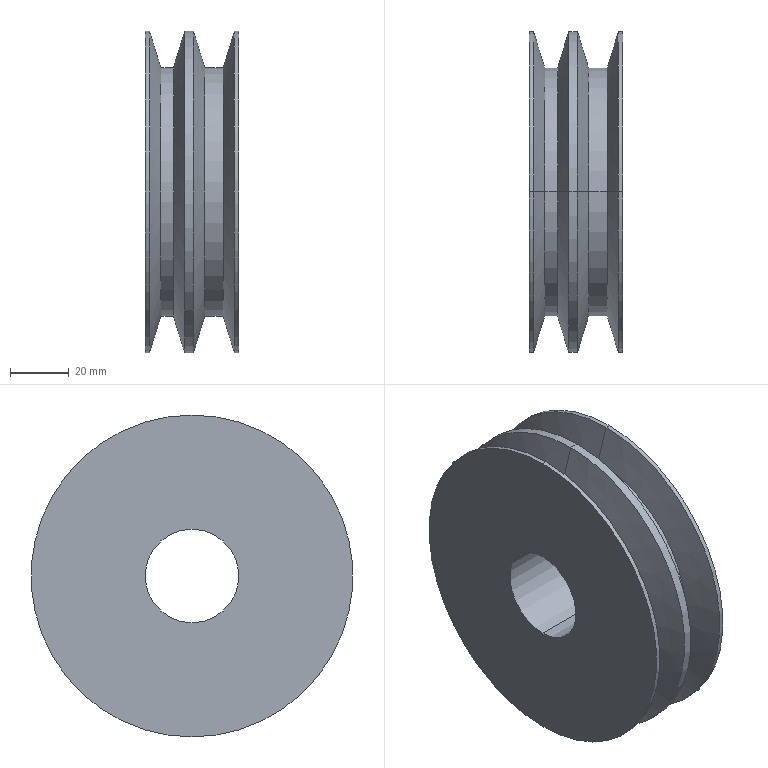Component | SolidWorks | TypeAPulley(Motor)-2 | 1 solid | 22 faces | box 32 x 110 x 110 mm | volume 206835 mm3 | cylinder 12 | cone 8 | plane 2 | commonest cylinder face diameters 110 x6 85 x4 32 x2
build123d program:
from build123d import *


with BuildPart() as part:
    # Sketch1 → Revolve1 (revolve)
    with BuildSketch(Plane.XY, mode=Mode.PRIVATE) as revolve1_sk:
        Polygon((0.4755, 16), (0.4755, 55), (1.975, 55), (5.797, 42.5), (10.154, 42.5), (13.975, 55), (16.975, 55), (20.797, 42.5), (27.154, 42.5), (30.975, 55), (32.475, 55), (32.475, 16), align=None)
    revolve(revolve1_sk.sketch.rotate(Axis((-58.13, 0, 0), (1, 0, 0)), 90), axis=Axis((-58.13, 0, 0), (1, 0, 0)))


solid = part.part

# Placed as in the assembly
solid = solid.moved(Location((-375.218, 1299.706, 687.116), (0, 0, 0)))
STEP:
#1=COLOUR_RGB('',0.7922,0.8196,0.9333);
#2=FILL_AREA_STYLE_COLOUR('',#1);
#3=FILL_AREA_STYLE('',(#2));
#4=SURFACE_STYLE_FILL_AREA(#3);
#5=SURFACE_SIDE_STYLE('',(#4));
#6=SURFACE_STYLE_USAGE(.BOTH.,#5);
#7=PRESENTATION_STYLE_ASSIGNMENT((#6));
#8=CARTESIAN_POINT('',(-13.954,51.17,28.725));
#9=VERTEX_POINT('',#8);
#10=CARTESIAN_POINT('',(-13.954,51.17,25.379));
#11=VERTEX_POINT('',#10);
#12=CARTESIAN_POINT('',(-13.954,51.17,27.052));
#13=DIRECTION('',(-1.,0.,0.));
#14=DIRECTION('',(0.,0.,1.));
#15=AXIS2_PLACEMENT_3D('',#12,#13,#14);
#16=CIRCLE('',#15,1.673);
#17=EDGE_CURVE('',#9,#11,#16,.T.);
#18=ORIENTED_EDGE('',*,*,#17,.T.);
#19=CARTESIAN_POINT('',(-14.104,51.17,24.886));
#20=VERTEX_POINT('',#19);
#21=CARTESIAN_POINT('',(-13.954,51.17,25.379));
#22=DIRECTION('',(-0.2924,0.,-0.9563));
#23=VECTOR('',#22,39.37);
#24=LINE('',#21,#23);
#25=EDGE_CURVE('',#11,#20,#24,.T.);
#26=ORIENTED_EDGE('',*,*,#25,.T.);
#27=CARTESIAN_POINT('',(-14.104,51.17,29.217));
#28=VERTEX_POINT('',#27);
#29=CARTESIAN_POINT('',(-14.104,51.17,27.052));
#30=DIRECTION('',(-1.,0.,0.));
#31=DIRECTION('',(0.,0.,1.));
#32=AXIS2_PLACEMENT_3D('',#29,#30,#31);
#33=CIRCLE('',#32,2.165);
#34=EDGE_CURVE('',#28,#20,#33,.T.);
#35=ORIENTED_EDGE('',*,*,#34,.F.);
#36=CARTESIAN_POINT('',(-13.954,51.17,28.725));
#37=DIRECTION('',(-0.2924,0.,0.9563));
#38=VECTOR('',#37,39.37);
#39=LINE('',#36,#38);
#40=EDGE_CURVE('',#9,#28,#39,.T.);
#41=ORIENTED_EDGE('',*,*,#40,.F.);
#42=EDGE_LOOP('',(#18,#26,#35,#41));
#43=FACE_OUTER_BOUND('',#42,.T.);
#44=CARTESIAN_POINT('',(-13.954,51.17,27.052));
#45=DIRECTION('',(-1.,0.,0.));
#46=DIRECTION('',(0.,0.,1.));
#47=AXIS2_PLACEMENT_3D('',#44,#45,#46);
#48=CONICAL_SURFACE('',#47,1.673,1.274);
#49=ADVANCED_FACE('',(#43),#48,.T.);
#50=ORIENTED_EDGE('',*,*,#34,.T.);
#51=CARTESIAN_POINT('',(-14.222,51.17,24.886));
#52=VERTEX_POINT('',#51);
#53=CARTESIAN_POINT('',(-17.061,51.17,24.886));
#54=DIRECTION('',(-1.,0.,0.));
#55=VECTOR('',#54,39.37);
#56=LINE('',#53,#55);
#57=EDGE_CURVE('',#20,#52,#56,.T.);
#58=ORIENTED_EDGE('',*,*,#57,.T.);
#59=CARTESIAN_POINT('',(-14.222,51.17,29.217));
#60=VERTEX_POINT('',#59);
#61=CARTESIAN_POINT('',(-14.222,51.17,27.052));
#62=DIRECTION('',(-1.,0.,0.));
#63=DIRECTION('',(0.,0.,1.));
#64=AXIS2_PLACEMENT_3D('',#61,#62,#63);
#65=CIRCLE('',#64,2.165);
#66=EDGE_CURVE('',#60,#52,#65,.T.);
#67=ORIENTED_EDGE('',*,*,#66,.F.);
#68=CARTESIAN_POINT('',(-17.061,51.17,29.217));
#69=DIRECTION('',(-1.,0.,0.));
#70=VECTOR('',#69,39.37);
#71=LINE('',#68,#70);
#72=EDGE_CURVE('',#28,#60,#71,.T.);
#73=ORIENTED_EDGE('',*,*,#72,.F.);
#74=EDGE_LOOP('',(#50,#58,#67,#73));
#75=FACE_OUTER_BOUND('',#74,.T.);
#76=CARTESIAN_POINT('',(-17.061,51.17,27.052));
#77=DIRECTION('',(-1.,0.,0.));
#78=DIRECTION('',(0.,0.,1.));
#79=AXIS2_PLACEMENT_3D('',#76,#77,#78);
#80=CYLINDRICAL_SURFACE('',#79,2.165);
#81=ADVANCED_FACE('',(#75),#80,.T.);
#82=CARTESIAN_POINT('',(-14.373,51.17,28.725));
#83=VERTEX_POINT('',#82);
#84=CARTESIAN_POINT('',(-14.373,51.17,25.379));
#85=VERTEX_POINT('',#84);
#86=CARTESIAN_POINT('',(-14.373,51.17,27.052));
#87=DIRECTION('',(-1.,0.,0.));
#88=DIRECTION('',(0.,0.,1.));
#89=AXIS2_PLACEMENT_3D('',#86,#87,#88);
#90=CIRCLE('',#89,1.673);
#91=EDGE_CURVE('',#83,#85,#90,.T.);
#92=ORIENTED_EDGE('',*,*,#91,.F.);
#93=CARTESIAN_POINT('',(-14.222,51.17,29.217));
#94=DIRECTION('',(0.2924,0.,0.9563));
#95=VECTOR('',#94,39.37);
#96=LINE('',#93,#95);
#97=EDGE_CURVE('',#83,#60,#96,.T.);
#98=ORIENTED_EDGE('',*,*,#97,.T.);
#99=ORIENTED_EDGE('',*,*,#66,.T.);
#100=CARTESIAN_POINT('',(-14.222,51.17,24.886));
#101=DIRECTION('',(0.2924,0.,-0.9563));
#102=VECTOR('',#101,39.37);
#103=LINE('',#100,#102);
#104=EDGE_CURVE('',#85,#52,#103,.T.);
#105=ORIENTED_EDGE('',*,*,#104,.F.);
#106=EDGE_LOOP('',(#92,#98,#99,#105));
#107=FACE_OUTER_BOUND('',#106,.T.);
#108=CARTESIAN_POINT('',(-14.222,51.17,27.052));
#109=DIRECTION('',(1.,0.,0.));
#110=DIRECTION('',(0.,0.,-1.));
#111=AXIS2_PLACEMENT_3D('',#108,#109,#110);
#112=CONICAL_SURFACE('',#111,2.165,1.274);
#113=ADVANCED_FACE('',(#107),#112,.T.);
#114=ORIENTED_EDGE('',*,*,#91,.T.);
#115=CARTESIAN_POINT('',(-14.544,51.17,25.379));
#116=VERTEX_POINT('',#115);
#117=CARTESIAN_POINT('',(-17.061,51.17,25.379));
#118=DIRECTION('',(-1.,0.,0.));
#119=VECTOR('',#118,39.37);
#120=LINE('',#117,#119);
#121=EDGE_CURVE('',#85,#116,#120,.T.);
#122=ORIENTED_EDGE('',*,*,#121,.T.);
#123=CARTESIAN_POINT('',(-14.544,51.17,28.725));
#124=VERTEX_POINT('',#123);
#125=CARTESIAN_POINT('',(-14.544,51.17,27.052));
#126=DIRECTION('',(-1.,0.,0.));
#127=DIRECTION('',(0.,0.,1.));
#128=AXIS2_PLACEMENT_3D('',#125,#126,#127);
#129=CIRCLE('',#128,1.673);
#130=EDGE_CURVE('',#124,#116,#129,.T.);
#131=ORIENTED_EDGE('',*,*,#130,.F.);
#132=CARTESIAN_POINT('',(-17.061,51.17,28.725));
#133=DIRECTION('',(-1.,0.,0.));
#134=VECTOR('',#133,39.37);
#135=LINE('',#132,#134);
#136=EDGE_CURVE('',#83,#124,#135,.T.);
#137=ORIENTED_EDGE('',*,*,#136,.F.);
#138=EDGE_LOOP('',(#114,#122,#131,#137));
#139=FACE_OUTER_BOUND('',#138,.T.);
#140=CARTESIAN_POINT('',(-17.061,51.17,27.052));
#141=DIRECTION('',(-1.,0.,0.));
#142=DIRECTION('',(0.,0.,1.));
#143=AXIS2_PLACEMENT_3D('',#140,#141,#142);
#144=CYLINDRICAL_SURFACE('',#143,1.673);
#145=ADVANCED_FACE('',(#139),#144,.T.);
#146=ORIENTED_EDGE('',*,*,#130,.T.);
#147=CARTESIAN_POINT('',(-14.695,51.17,24.886));
#148=VERTEX_POINT('',#147);
#149=CARTESIAN_POINT('',(-14.544,51.17,25.379));
#150=DIRECTION('',(-0.2924,0.,-0.9563));
#151=VECTOR('',#150,39.37);
#152=LINE('',#149,#151);
#153=EDGE_CURVE('',#116,#148,#152,.T.);
#154=ORIENTED_EDGE('',*,*,#153,.T.);
#155=CARTESIAN_POINT('',(-14.695,51.17,29.217));
#156=VERTEX_POINT('',#155);
#157=CARTESIAN_POINT('',(-14.695,51.17,27.052));
#158=DIRECTION('',(-1.,0.,0.));
#159=DIRECTION('',(0.,0.,1.));
#160=AXIS2_PLACEMENT_3D('',#157,#158,#159);
#161=CIRCLE('',#160,2.165);
#162=EDGE_CURVE('',#156,#148,#161,.T.);
#163=ORIENTED_EDGE('',*,*,#162,.F.);
#164=CARTESIAN_POINT('',(-14.544,51.17,28.725));
#165=DIRECTION('',(-0.2924,0.,0.9563));
#166=VECTOR('',#165,39.37);
#167=LINE('',#164,#166);
#168=EDGE_CURVE('',#124,#156,#167,.T.);
#169=ORIENTED_EDGE('',*,*,#168,.F.);
#170=EDGE_LOOP('',(#146,#154,#163,#169));
#171=FACE_OUTER_BOUND('',#170,.T.);
#172=CARTESIAN_POINT('',(-14.544,51.17,27.052));
#173=DIRECTION('',(-1.,0.,0.));
#174=DIRECTION('',(0.,0.,1.));
#175=AXIS2_PLACEMENT_3D('',#172,#173,#174);
#176=CONICAL_SURFACE('',#175,1.673,1.274);
#177=ADVANCED_FACE('',(#171),#176,.T.);
#178=ORIENTED_EDGE('',*,*,#162,.T.);
#179=CARTESIAN_POINT('',(-14.754,51.17,24.886));
#180=VERTEX_POINT('',#179);
#181=CARTESIAN_POINT('',(-17.061,51.17,24.886));
#182=DIRECTION('',(-1.,0.,0.));
#183=VECTOR('',#182,39.37);
#184=LINE('',#181,#183);
#185=EDGE_CURVE('',#148,#180,#184,.T.);
#186=ORIENTED_EDGE('',*,*,#185,.T.);
#187=CARTESIAN_POINT('',(-14.754,51.17,29.217));
#188=VERTEX_POINT('',#187);
#189=CARTESIAN_POINT('',(-14.754,51.17,27.052));
#190=DIRECTION('',(-1.,0.,0.));
#191=DIRECTION('',(0.,0.,1.));
#192=AXIS2_PLACEMENT_3D('',#189,#190,#191);
#193=CIRCLE('',#192,2.165);
#194=EDGE_CURVE('',#188,#180,#193,.T.);
#195=ORIENTED_EDGE('',*,*,#194,.F.);
#196=CARTESIAN_POINT('',(-17.061,51.17,29.217));
#197=DIRECTION('',(-1.,0.,0.));
#198=VECTOR('',#197,39.37);
#199=LINE('',#196,#198);
#200=EDGE_CURVE('',#156,#188,#199,.T.);
#201=ORIENTED_EDGE('',*,*,#200,.F.);
#202=EDGE_LOOP('',(#178,#186,#195,#201));
#203=FACE_OUTER_BOUND('',#202,.T.);
#204=CARTESIAN_POINT('',(-17.061,51.17,27.052));
#205=DIRECTION('',(-1.,0.,0.));
#206=DIRECTION('',(0.,0.,1.));
#207=AXIS2_PLACEMENT_3D('',#204,#205,#206);
#208=CYLINDRICAL_SURFACE('',#207,2.165);
#209=ADVANCED_FACE('',(#203),#208,.T.);
#210=CARTESIAN_POINT('',(-13.494,51.17,26.422));
#211=VERTEX_POINT('',#210);
#212=CARTESIAN_POINT('',(-13.494,51.17,27.682));
#213=VERTEX_POINT('',#212);
#214=CARTESIAN_POINT('',(-13.494,51.17,27.052));
#215=DIRECTION('',(-1.,0.,0.));
#216=DIRECTION('',(0.,0.,1.));
#217=AXIS2_PLACEMENT_3D('',#214,#215,#216);
#218=CIRCLE('',#217,0.6299);
#219=EDGE_CURVE('',#211,#213,#218,.T.);
#220=ORIENTED_EDGE('',*,*,#219,.F.);
#221=CARTESIAN_POINT('',(-14.754,51.17,26.422));
#222=VERTEX_POINT('',#221);
#223=CARTESIAN_POINT('',(-17.061,51.17,26.422));
#224=DIRECTION('',(-1.,0.,0.));
#225=VECTOR('',#224,39.37);
#226=LINE('',#223,#225);
#227=EDGE_CURVE('',#211,#222,#226,.T.);
#228=ORIENTED_EDGE('',*,*,#227,.T.);
#229=CARTESIAN_POINT('',(-14.754,51.17,27.682));
#230=VERTEX_POINT('',#229);
#231=CARTESIAN_POINT('',(-14.754,51.17,27.052));
#232=DIRECTION('',(-1.,0.,0.));
#233=DIRECTION('',(0.,0.,1.));
#234=AXIS2_PLACEMENT_3D('',#231,#232,#233);
#235=CIRCLE('',#234,0.6299);
#236=EDGE_CURVE('',#222,#230,#235,.T.);
#237=ORIENTED_EDGE('',*,*,#236,.T.);
#238=CARTESIAN_POINT('',(-17.061,51.17,27.682));
#239=DIRECTION('',(-1.,0.,0.));
#240=VECTOR('',#239,39.37);
#241=LINE('',#238,#240);
#242=EDGE_CURVE('',#213,#230,#241,.T.);
#243=ORIENTED_EDGE('',*,*,#242,.F.);
#244=EDGE_LOOP('',(#220,#228,#237,#243));
#245=FACE_OUTER_BOUND('',#244,.T.);
#246=CARTESIAN_POINT('',(-17.061,51.17,27.052));
#247=DIRECTION('',(-1.,0.,0.));
#248=DIRECTION('',(0.,0.,1.));
#249=AXIS2_PLACEMENT_3D('',#246,#247,#248);
#250=CYLINDRICAL_SURFACE('',#249,0.6299);
#251=ADVANCED_FACE('',(#245),#250,.F.);
#252=CARTESIAN_POINT('',(-13.494,51.17,29.217));
#253=VERTEX_POINT('',#252);
#254=CARTESIAN_POINT('',(-13.494,51.17,24.886));
#255=VERTEX_POINT('',#254);
#256=CARTESIAN_POINT('',(-13.494,51.17,27.052));
#257=DIRECTION('',(-1.,0.,0.));
#258=DIRECTION('',(0.,0.,1.));
#259=AXIS2_PLACEMENT_3D('',#256,#257,#258);
#260=CIRCLE('',#259,2.165);
#261=EDGE_CURVE('',#253,#255,#260,.T.);
#262=ORIENTED_EDGE('',*,*,#261,.T.);
#263=CARTESIAN_POINT('',(-13.553,51.17,24.886));
#264=VERTEX_POINT('',#263);
#265=CARTESIAN_POINT('',(-17.061,51.17,24.886));
#266=DIRECTION('',(-1.,0.,0.));
#267=VECTOR('',#266,39.37);
#268=LINE('',#265,#267);
#269=EDGE_CURVE('',#255,#264,#268,.T.);
#270=ORIENTED_EDGE('',*,*,#269,.T.);
#271=CARTESIAN_POINT('',(-13.553,51.17,29.217));
#272=VERTEX_POINT('',#271);
#273=CARTESIAN_POINT('',(-13.553,51.17,27.052));
#274=DIRECTION('',(-1.,0.,0.));
#275=DIRECTION('',(0.,0.,1.));
#276=AXIS2_PLACEMENT_3D('',#273,#274,#275);
#277=CIRCLE('',#276,2.165);
#278=EDGE_CURVE('',#272,#264,#277,.T.);
#279=ORIENTED_EDGE('',*,*,#278,.F.);
#280=CARTESIAN_POINT('',(-17.061,51.17,29.217));
#281=DIRECTION('',(-1.,0.,0.));
#282=VECTOR('',#281,39.37);
#283=LINE('',#280,#282);
#284=EDGE_CURVE('',#253,#272,#283,.T.);
#285=ORIENTED_EDGE('',*,*,#284,.F.);
#286=EDGE_LOOP('',(#262,#270,#279,#285));
#287=FACE_OUTER_BOUND('',#286,.T.);
#288=CARTESIAN_POINT('',(-17.061,51.17,27.052));
#289=DIRECTION('',(-1.,0.,0.));
#290=DIRECTION('',(0.,0.,1.));
#291=AXIS2_PLACEMENT_3D('',#288,#289,#290);
#292=CYLINDRICAL_SURFACE('',#291,2.165);
#293=ADVANCED_FACE('',(#287),#292,.T.);
#294=CARTESIAN_POINT('',(-13.703,51.17,28.725));
#295=VERTEX_POINT('',#294);
#296=CARTESIAN_POINT('',(-13.703,51.17,25.379));
#297=VERTEX_POINT('',#296);
#298=CARTESIAN_POINT('',(-13.703,51.17,27.052));
#299=DIRECTION('',(-1.,0.,0.));
#300=DIRECTION('',(0.,0.,1.));
#301=AXIS2_PLACEMENT_3D('',#298,#299,#300);
#302=CIRCLE('',#301,1.673);
#303=EDGE_CURVE('',#295,#297,#302,.T.);
#304=ORIENTED_EDGE('',*,*,#303,.F.);
#305=CARTESIAN_POINT('',(-13.553,51.17,29.217));
#306=DIRECTION('',(0.2924,0.,0.9563));
#307=VECTOR('',#306,39.37);
#308=LINE('',#305,#307);
#309=EDGE_CURVE('',#295,#272,#308,.T.);
#310=ORIENTED_EDGE('',*,*,#309,.T.);
#311=ORIENTED_EDGE('',*,*,#278,.T.);
#312=CARTESIAN_POINT('',(-13.553,51.17,24.886));
#313=DIRECTION('',(0.2924,0.,-0.9563));
#314=VECTOR('',#313,39.37);
#315=LINE('',#312,#314);
#316=EDGE_CURVE('',#297,#264,#315,.T.);
#317=ORIENTED_EDGE('',*,*,#316,.F.);
#318=EDGE_LOOP('',(#304,#310,#311,#317));
#319=FACE_OUTER_BOUND('',#318,.T.);
#320=CARTESIAN_POINT('',(-13.553,51.17,27.052));
#321=DIRECTION('',(1.,0.,0.));
#322=DIRECTION('',(0.,0.,-1.));
#323=AXIS2_PLACEMENT_3D('',#320,#321,#322);
#324=CONICAL_SURFACE('',#323,2.165,1.274);
#325=ADVANCED_FACE('',(#319),#324,.T.);
#326=ORIENTED_EDGE('',*,*,#303,.T.);
#327=CARTESIAN_POINT('',(-17.061,51.17,25.379));
#328=DIRECTION('',(-1.,0.,0.));
#329=VECTOR('',#328,39.37);
#330=LINE('',#327,#329);
#331=EDGE_CURVE('',#297,#11,#330,.T.);
#332=ORIENTED_EDGE('',*,*,#331,.T.);
#333=ORIENTED_EDGE('',*,*,#17,.F.);
#334=CARTESIAN_POINT('',(-17.061,51.17,28.725));
#335=DIRECTION('',(-1.,0.,0.));
#336=VECTOR('',#335,39.37);
#337=LINE('',#334,#336);
#338=EDGE_CURVE('',#295,#9,#337,.T.);
#339=ORIENTED_EDGE('',*,*,#338,.F.);
#340=EDGE_LOOP('',(#326,#332,#333,#339));
#341=FACE_OUTER_BOUND('',#340,.T.);
#342=CARTESIAN_POINT('',(-17.061,51.17,27.052));
#343=DIRECTION('',(-1.,0.,0.));
#344=DIRECTION('',(0.,0.,1.));
#345=AXIS2_PLACEMENT_3D('',#342,#343,#344);
#346=CYLINDRICAL_SURFACE('',#345,1.673);
#347=ADVANCED_FACE('',(#341),#346,.T.);
#348=ORIENTED_EDGE('',*,*,#331,.F.);
#349=CARTESIAN_POINT('',(-13.703,51.17,27.052));
#350=DIRECTION('',(-1.,0.,0.));
#351=DIRECTION('',(0.,0.,1.));
#352=AXIS2_PLACEMENT_3D('',#349,#350,#351);
#353=CIRCLE('',#352,1.673);
#354=EDGE_CURVE('',#297,#295,#353,.T.);
#355=ORIENTED_EDGE('',*,*,#354,.T.);
#356=ORIENTED_EDGE('',*,*,#338,.T.);
#357=CARTESIAN_POINT('',(-13.954,51.17,27.052));
#358=DIRECTION('',(-1.,0.,0.));
#359=DIRECTION('',(0.,0.,1.));
#360=AXIS2_PLACEMENT_3D('',#357,#358,#359);
#361=CIRCLE('',#360,1.673);
#362=EDGE_CURVE('',#11,#9,#361,.T.);
#363=ORIENTED_EDGE('',*,*,#362,.F.);
#364=EDGE_LOOP('',(#348,#355,#356,#363));
#365=FACE_OUTER_BOUND('',#364,.T.);
#366=CARTESIAN_POINT('',(-17.061,51.17,27.052));
#367=DIRECTION('',(-1.,0.,0.));
#368=DIRECTION('',(0.,0.,1.));
#369=AXIS2_PLACEMENT_3D('',#366,#367,#368);
#370=CYLINDRICAL_SURFACE('',#369,1.673);
#371=ADVANCED_FACE('',(#365),#370,.T.);
#372=ORIENTED_EDGE('',*,*,#309,.F.);
#373=ORIENTED_EDGE('',*,*,#354,.F.);
#374=ORIENTED_EDGE('',*,*,#316,.T.);
#375=CARTESIAN_POINT('',(-13.553,51.17,27.052));
#376=DIRECTION('',(-1.,0.,0.));
#377=DIRECTION('',(0.,0.,1.));
#378=AXIS2_PLACEMENT_3D('',#375,#376,#377);
#379=CIRCLE('',#378,2.165);
#380=EDGE_CURVE('',#264,#272,#379,.T.);
#381=ORIENTED_EDGE('',*,*,#380,.T.);
#382=EDGE_LOOP('',(#372,#373,#374,#381));
#383=FACE_OUTER_BOUND('',#382,.T.);
#384=CARTESIAN_POINT('',(-13.553,51.17,27.052));
#385=DIRECTION('',(1.,0.,0.));
#386=DIRECTION('',(0.,0.,-1.));
#387=AXIS2_PLACEMENT_3D('',#384,#385,#386);
#388=CONICAL_SURFACE('',#387,2.165,1.274);
#389=ADVANCED_FACE('',(#383),#388,.T.);
#390=ORIENTED_EDGE('',*,*,#269,.F.);
#391=CARTESIAN_POINT('',(-13.494,51.17,27.052));
#392=DIRECTION('',(-1.,0.,0.));
#393=DIRECTION('',(0.,0.,1.));
#394=AXIS2_PLACEMENT_3D('',#391,#392,#393);
#395=CIRCLE('',#394,2.165);
#396=EDGE_CURVE('',#255,#253,#395,.T.);
#397=ORIENTED_EDGE('',*,*,#396,.T.);
#398=ORIENTED_EDGE('',*,*,#284,.T.);
#399=ORIENTED_EDGE('',*,*,#380,.F.);
#400=EDGE_LOOP('',(#390,#397,#398,#399));
#401=FACE_OUTER_BOUND('',#400,.T.);
#402=CARTESIAN_POINT('',(-17.061,51.17,27.052));
#403=DIRECTION('',(-1.,0.,0.));
#404=DIRECTION('',(0.,0.,1.));
#405=AXIS2_PLACEMENT_3D('',#402,#403,#404);
#406=CYLINDRICAL_SURFACE('',#405,2.165);
#407=ADVANCED_FACE('',(#401),#406,.T.);
#408=ORIENTED_EDGE('',*,*,#261,.F.);
#409=ORIENTED_EDGE('',*,*,#396,.F.);
#410=EDGE_LOOP('',(#408,#409));
#411=FACE_OUTER_BOUND('',#410,.T.);
#412=CARTESIAN_POINT('',(-13.494,51.17,27.052));
#413=DIRECTION('',(-1.,0.,0.));
#414=DIRECTION('',(0.,0.,1.));
#415=AXIS2_PLACEMENT_3D('',#412,#413,#414);
#416=CIRCLE('',#415,0.6299);
#417=EDGE_CURVE('',#213,#211,#416,.T.);
#418=ORIENTED_EDGE('',*,*,#417,.T.);
#419=ORIENTED_EDGE('',*,*,#219,.T.);
#420=EDGE_LOOP('',(#418,#419));
#421=FACE_BOUND('',#420,.T.);
#422=CARTESIAN_POINT('',(-13.494,53.335,27.052));
#423=DIRECTION('',(-1.,0.,0.));
#424=DIRECTION('',(0.,0.,1.));
#425=AXIS2_PLACEMENT_3D('',#422,#423,#424);
#426=PLANE('',#425);
#427=ADVANCED_FACE('',(#411,#421),#426,.F.);
#428=ORIENTED_EDGE('',*,*,#227,.F.);
#429=ORIENTED_EDGE('',*,*,#417,.F.);
#430=ORIENTED_EDGE('',*,*,#242,.T.);
#431=CARTESIAN_POINT('',(-14.754,51.17,27.052));
#432=DIRECTION('',(-1.,0.,0.));
#433=DIRECTION('',(0.,0.,1.));
#434=AXIS2_PLACEMENT_3D('',#431,#432,#433);
#435=CIRCLE('',#434,0.6299);
#436=EDGE_CURVE('',#230,#222,#435,.T.);
#437=ORIENTED_EDGE('',*,*,#436,.T.);
#438=EDGE_LOOP('',(#428,#429,#430,#437));
#439=FACE_OUTER_BOUND('',#438,.T.);
#440=CARTESIAN_POINT('',(-17.061,51.17,27.052));
#441=DIRECTION('',(-1.,0.,0.));
#442=DIRECTION('',(0.,0.,1.));
#443=AXIS2_PLACEMENT_3D('',#440,#441,#442);
#444=CYLINDRICAL_SURFACE('',#443,0.6299);
#445=ADVANCED_FACE('',(#439),#444,.F.);
#446=ORIENTED_EDGE('',*,*,#436,.F.);
#447=ORIENTED_EDGE('',*,*,#236,.F.);
#448=EDGE_LOOP('',(#446,#447));
#449=FACE_BOUND('',#448,.T.);
#450=ORIENTED_EDGE('',*,*,#194,.T.);
#451=CARTESIAN_POINT('',(-14.754,51.17,27.052));
#452=DIRECTION('',(-1.,0.,0.));
#453=DIRECTION('',(0.,0.,1.));
#454=AXIS2_PLACEMENT_3D('',#451,#452,#453);
#455=CIRCLE('',#454,2.165);
#456=EDGE_CURVE('',#180,#188,#455,.T.);
#457=ORIENTED_EDGE('',*,*,#456,.T.);
#458=EDGE_LOOP('',(#450,#457));
#459=FACE_OUTER_BOUND('',#458,.T.);
#460=CARTESIAN_POINT('',(-14.754,51.799,27.052));
#461=DIRECTION('',(1.,0.,0.));
#462=DIRECTION('',(0.,0.,-1.));
#463=AXIS2_PLACEMENT_3D('',#460,#461,#462);
#464=PLANE('',#463);
#465=ADVANCED_FACE('',(#449,#459),#464,.F.);
#466=ORIENTED_EDGE('',*,*,#185,.F.);
#467=CARTESIAN_POINT('',(-14.695,51.17,27.052));
#468=DIRECTION('',(-1.,0.,0.));
#469=DIRECTION('',(0.,0.,1.));
#470=AXIS2_PLACEMENT_3D('',#467,#468,#469);
#471=CIRCLE('',#470,2.165);
#472=EDGE_CURVE('',#148,#156,#471,.T.);
#473=ORIENTED_EDGE('',*,*,#472,.T.);
#474=ORIENTED_EDGE('',*,*,#200,.T.);
#475=ORIENTED_EDGE('',*,*,#456,.F.);
#476=EDGE_LOOP('',(#466,#473,#474,#475));
#477=FACE_OUTER_BOUND('',#476,.T.);
#478=CARTESIAN_POINT('',(-17.061,51.17,27.052));
#479=DIRECTION('',(-1.,0.,0.));
#480=DIRECTION('',(0.,0.,1.));
#481=AXIS2_PLACEMENT_3D('',#478,#479,#480);
#482=CYLINDRICAL_SURFACE('',#481,2.165);
#483=ADVANCED_FACE('',(#477),#482,.T.);
#484=ORIENTED_EDGE('',*,*,#153,.F.);
#485=CARTESIAN_POINT('',(-14.544,51.17,27.052));
#486=DIRECTION('',(-1.,0.,0.));
#487=DIRECTION('',(0.,0.,1.));
#488=AXIS2_PLACEMENT_3D('',#485,#486,#487);
#489=CIRCLE('',#488,1.673);
#490=EDGE_CURVE('',#116,#124,#489,.T.);
#491=ORIENTED_EDGE('',*,*,#490,.T.);
#492=ORIENTED_EDGE('',*,*,#168,.T.);
#493=ORIENTED_EDGE('',*,*,#472,.F.);
#494=EDGE_LOOP('',(#484,#491,#492,#493));
#495=FACE_OUTER_BOUND('',#494,.T.);
#496=CARTESIAN_POINT('',(-14.544,51.17,27.052));
#497=DIRECTION('',(-1.,0.,0.));
#498=DIRECTION('',(0.,0.,1.));
#499=AXIS2_PLACEMENT_3D('',#496,#497,#498);
#500=CONICAL_SURFACE('',#499,1.673,1.274);
#501=ADVANCED_FACE('',(#495),#500,.T.);
#502=ORIENTED_EDGE('',*,*,#121,.F.);
#503=CARTESIAN_POINT('',(-14.373,51.17,27.052));
#504=DIRECTION('',(-1.,0.,0.));
#505=DIRECTION('',(0.,0.,1.));
#506=AXIS2_PLACEMENT_3D('',#503,#504,#505);
#507=CIRCLE('',#506,1.673);
#508=EDGE_CURVE('',#85,#83,#507,.T.);
#509=ORIENTED_EDGE('',*,*,#508,.T.);
#510=ORIENTED_EDGE('',*,*,#136,.T.);
#511=ORIENTED_EDGE('',*,*,#490,.F.);
#512=EDGE_LOOP('',(#502,#509,#510,#511));
#513=FACE_OUTER_BOUND('',#512,.T.);
#514=CARTESIAN_POINT('',(-17.061,51.17,27.052));
#515=DIRECTION('',(-1.,0.,0.));
#516=DIRECTION('',(0.,0.,1.));
#517=AXIS2_PLACEMENT_3D('',#514,#515,#516);
#518=CYLINDRICAL_SURFACE('',#517,1.673);
#519=ADVANCED_FACE('',(#513),#518,.T.);
#520=ORIENTED_EDGE('',*,*,#97,.F.);
#521=ORIENTED_EDGE('',*,*,#508,.F.);
#522=ORIENTED_EDGE('',*,*,#104,.T.);
#523=CARTESIAN_POINT('',(-14.222,51.17,27.052));
#524=DIRECTION('',(-1.,0.,0.));
#525=DIRECTION('',(0.,0.,1.));
#526=AXIS2_PLACEMENT_3D('',#523,#524,#525);
#527=CIRCLE('',#526,2.165);
#528=EDGE_CURVE('',#52,#60,#527,.T.);
#529=ORIENTED_EDGE('',*,*,#528,.T.);
#530=EDGE_LOOP('',(#520,#521,#522,#529));
#531=FACE_OUTER_BOUND('',#530,.T.);
#532=CARTESIAN_POINT('',(-14.222,51.17,27.052));
#533=DIRECTION('',(1.,0.,0.));
#534=DIRECTION('',(0.,0.,-1.));
#535=AXIS2_PLACEMENT_3D('',#532,#533,#534);
#536=CONICAL_SURFACE('',#535,2.165,1.274);
#537=ADVANCED_FACE('',(#531),#536,.T.);
#538=ORIENTED_EDGE('',*,*,#57,.F.);
#539=CARTESIAN_POINT('',(-14.104,51.17,27.052));
#540=DIRECTION('',(-1.,0.,0.));
#541=DIRECTION('',(0.,0.,1.));
#542=AXIS2_PLACEMENT_3D('',#539,#540,#541);
#543=CIRCLE('',#542,2.165);
#544=EDGE_CURVE('',#20,#28,#543,.T.);
#545=ORIENTED_EDGE('',*,*,#544,.T.);
#546=ORIENTED_EDGE('',*,*,#72,.T.);
#547=ORIENTED_EDGE('',*,*,#528,.F.);
#548=EDGE_LOOP('',(#538,#545,#546,#547));
#549=FACE_OUTER_BOUND('',#548,.T.);
#550=CARTESIAN_POINT('',(-17.061,51.17,27.052));
#551=DIRECTION('',(-1.,0.,0.));
#552=DIRECTION('',(0.,0.,1.));
#553=AXIS2_PLACEMENT_3D('',#550,#551,#552);
#554=CYLINDRICAL_SURFACE('',#553,2.165);
#555=ADVANCED_FACE('',(#549),#554,.T.);
#556=ORIENTED_EDGE('',*,*,#25,.F.);
#557=ORIENTED_EDGE('',*,*,#362,.T.);
#558=ORIENTED_EDGE('',*,*,#40,.T.);
#559=ORIENTED_EDGE('',*,*,#544,.F.);
#560=EDGE_LOOP('',(#556,#557,#558,#559));
#561=FACE_OUTER_BOUND('',#560,.T.);
#562=CARTESIAN_POINT('',(-13.954,51.17,27.052));
#563=DIRECTION('',(-1.,0.,0.));
#564=DIRECTION('',(0.,0.,1.));
#565=AXIS2_PLACEMENT_3D('',#562,#563,#564);
#566=CONICAL_SURFACE('',#565,1.673,1.274);
#567=ADVANCED_FACE('',(#561),#566,.T.);
#568=CLOSED_SHELL('',(#49,#81,#113,#145,#177,#209,#251,#293,#325,#347,#371,#389,#407,#427,#445,#465,#483,#501,#519,#537,#555,#567));
#569=MANIFOLD_SOLID_BREP('',#568);
#570=STYLED_ITEM('',(#7),#569);
#571=(LENGTH_UNIT()NAMED_UNIT(*)SI_UNIT($,.METRE.));
#572=LENGTH_MEASURE_WITH_UNIT(LENGTH_MEASURE(0.0254),#571);
#573=DIMENSIONAL_EXPONENTS(1.,0.,0.,0.,0.,0.,0.);
#574=(CONVERSION_BASED_UNIT('',#572)LENGTH_UNIT()NAMED_UNIT(#573));
#575=UNCERTAINTY_MEASURE_WITH_UNIT(LENGTH_MEASURE(0.00001),#574,'','');
#576=(NAMED_UNIT(*)PLANE_ANGLE_UNIT()SI_UNIT($,.RADIAN.));
#577=(NAMED_UNIT(*)SI_UNIT($,.STERADIAN.)SOLID_ANGLE_UNIT());
#578=(GEOMETRIC_REPRESENTATION_CONTEXT(3)GLOBAL_UNCERTAINTY_ASSIGNED_CONTEXT((#575))GLOBAL_UNIT_ASSIGNED_CONTEXT((#574,#576,#577))REPRESENTATION_CONTEXT('',''));
#579=MECHANICAL_DESIGN_GEOMETRIC_PRESENTATION_REPRESENTATION('',(#570),#578);
#580=PRESENTATION_LAYER_ASSIGNMENT('','',(#570));
#581=CARTESIAN_POINT('',(0.,0.,0.));
#582=DIRECTION('',(0.,0.,1.));
#583=DIRECTION('',(1.,0.,0.));
#584=AXIS2_PLACEMENT_3D('',#581,#582,#583);
#585=(LENGTH_UNIT()NAMED_UNIT(*)SI_UNIT($,.METRE.));
#586=LENGTH_MEASURE_WITH_UNIT(LENGTH_MEASURE(0.0254),#585);
#587=DIMENSIONAL_EXPONENTS(1.,0.,0.,0.,0.,0.,0.);
#588=(CONVERSION_BASED_UNIT('',#586)LENGTH_UNIT()NAMED_UNIT(#587));
#589=UNCERTAINTY_MEASURE_WITH_UNIT(LENGTH_MEASURE(0.00001),#588,'','');
#590=(NAMED_UNIT(*)PLANE_ANGLE_UNIT()SI_UNIT($,.RADIAN.));
#591=(NAMED_UNIT(*)SI_UNIT($,.STERADIAN.)SOLID_ANGLE_UNIT());
#592=(GEOMETRIC_REPRESENTATION_CONTEXT(3)GLOBAL_UNCERTAINTY_ASSIGNED_CONTEXT((#589))GLOBAL_UNIT_ASSIGNED_CONTEXT((#588,#590,#591))REPRESENTATION_CONTEXT('',''));
#593=ADVANCED_BREP_SHAPE_REPRESENTATION('',(#569,#584),#592);